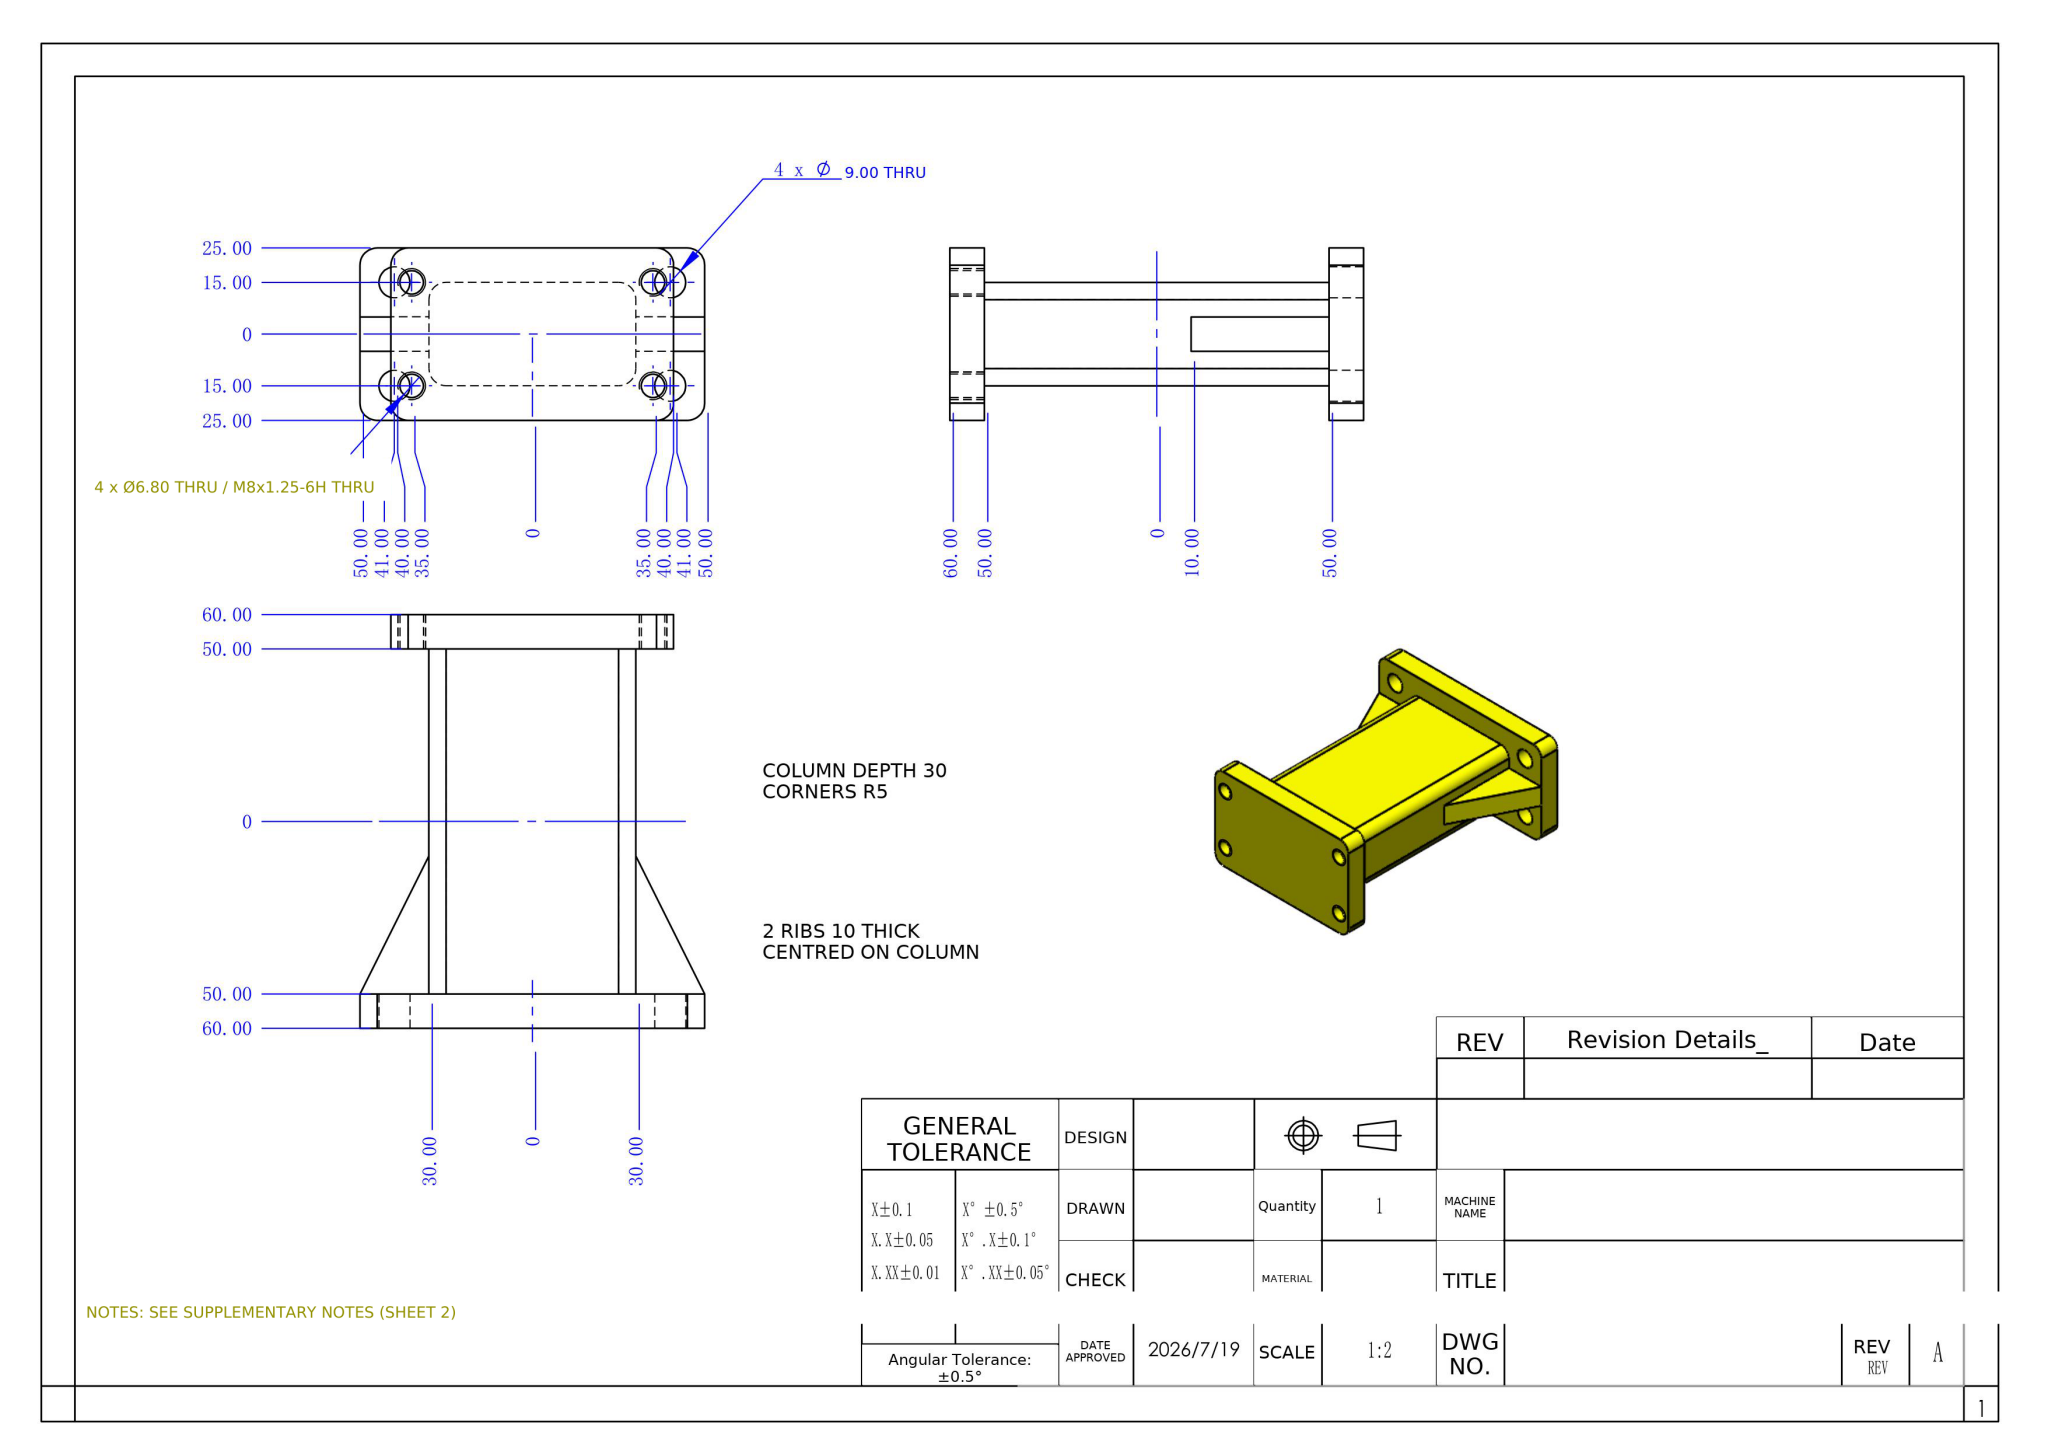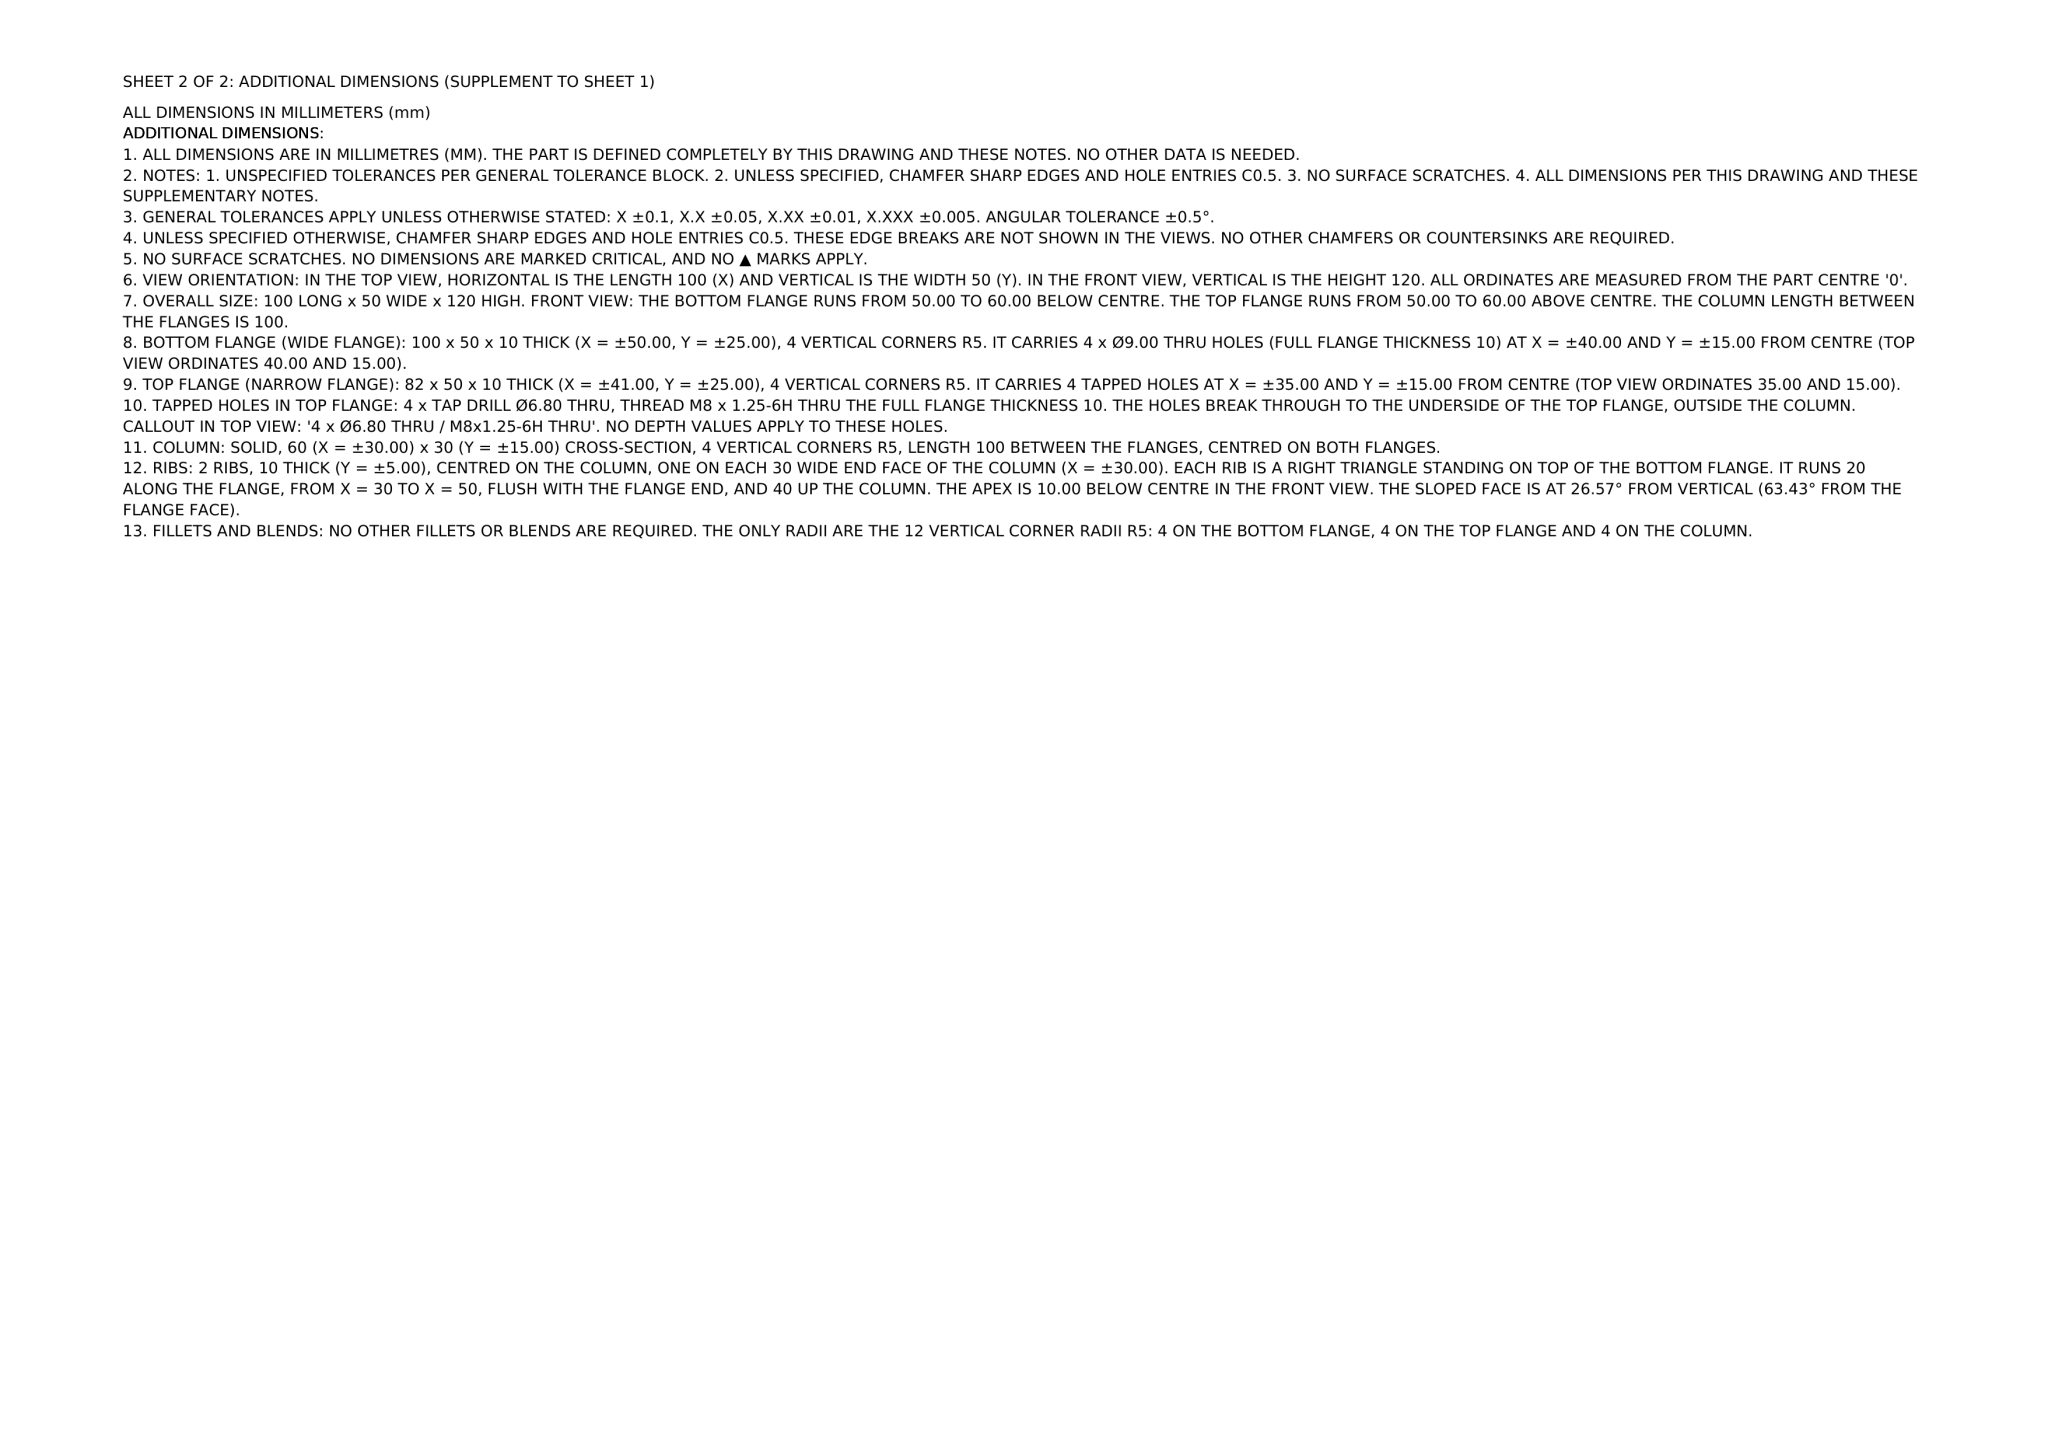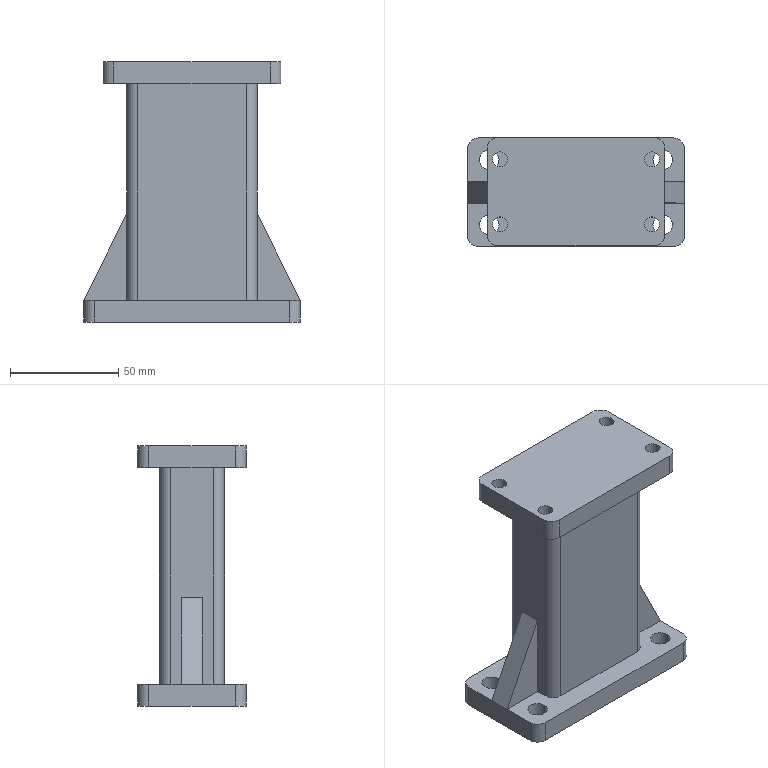Part | NX | mm | 1 solid | 51 faces | box 100 x 50 x 120 mm | volume 272427 mm3 | cylinder 28 | plane 23 | commonest cylinder face diameters 10 x12 6.8 x8 9 x8